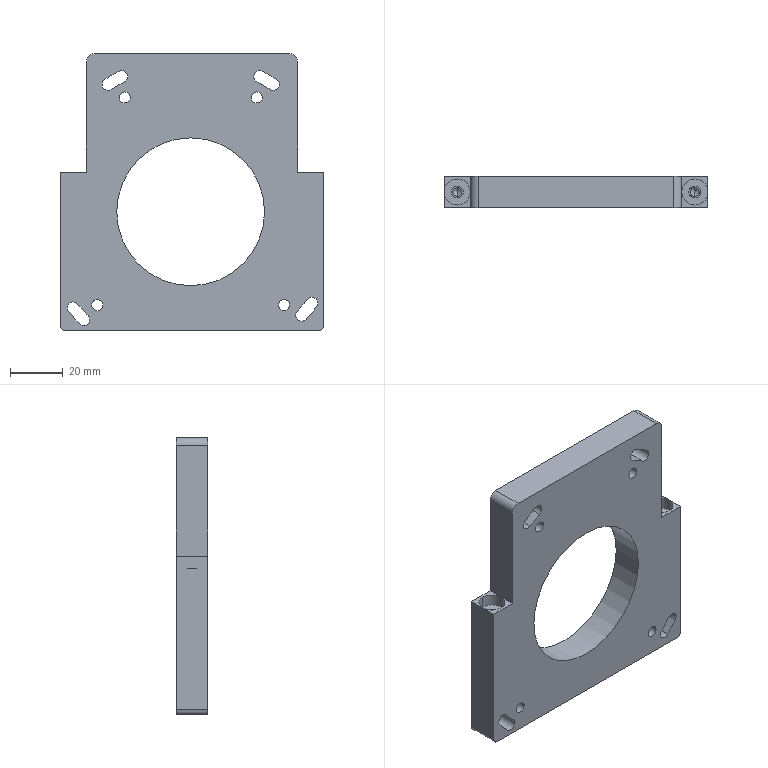CAM job | Mastercam | mm | 14 operations | part box 100 x 11.9 x 105
1. Facing | 24 - 100 平铣刀
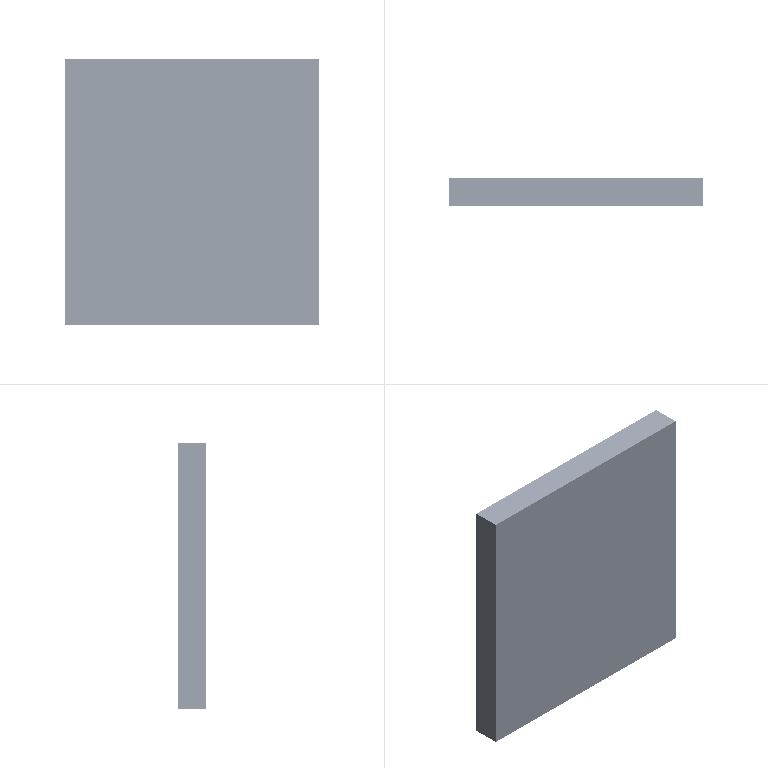2. 2D High Speed (2D Dynamic Mill) | 9 - 10 平铣刀
3. 2D High Speed (2D Dynamic Mill) | 9 - 10 平铣刀
4. Contour (Ramp) | 3 - 3 平铣刀
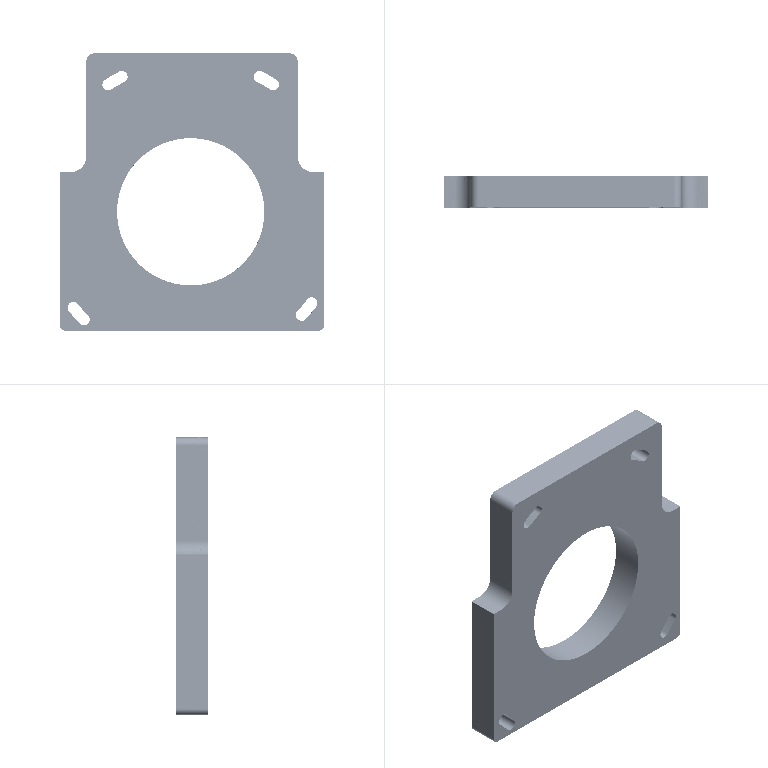5. Contour (Ramp) | 3 - 3 平铣刀
6. Contour (2D) | 10 - 10 平铣刀
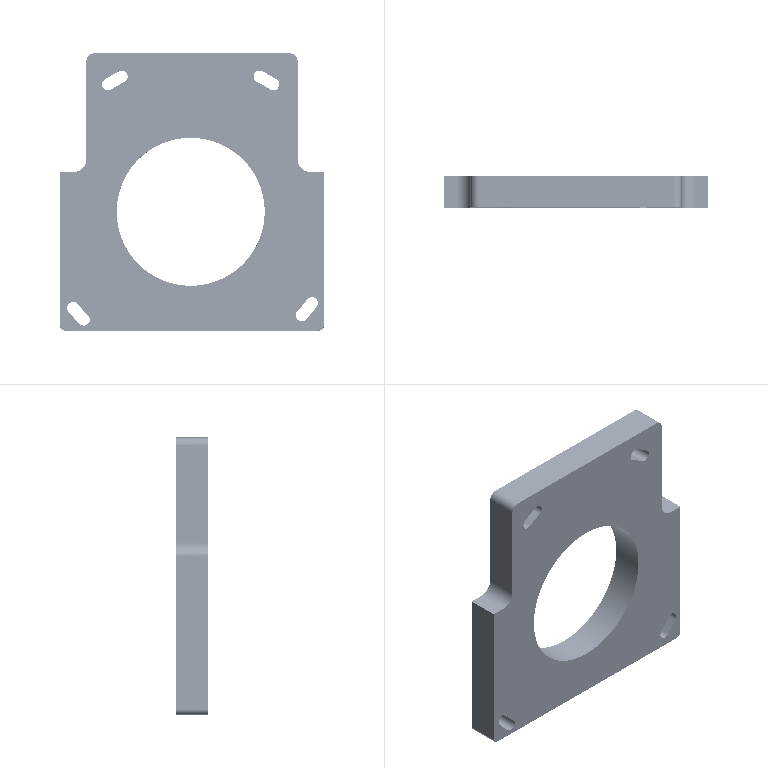7. Contour (2D chamfer) | 5 - 4 倒角刀
8. Facing | 24 - 100 平铣刀
9. Contour (2D chamfer) | 5 - 4 倒角刀
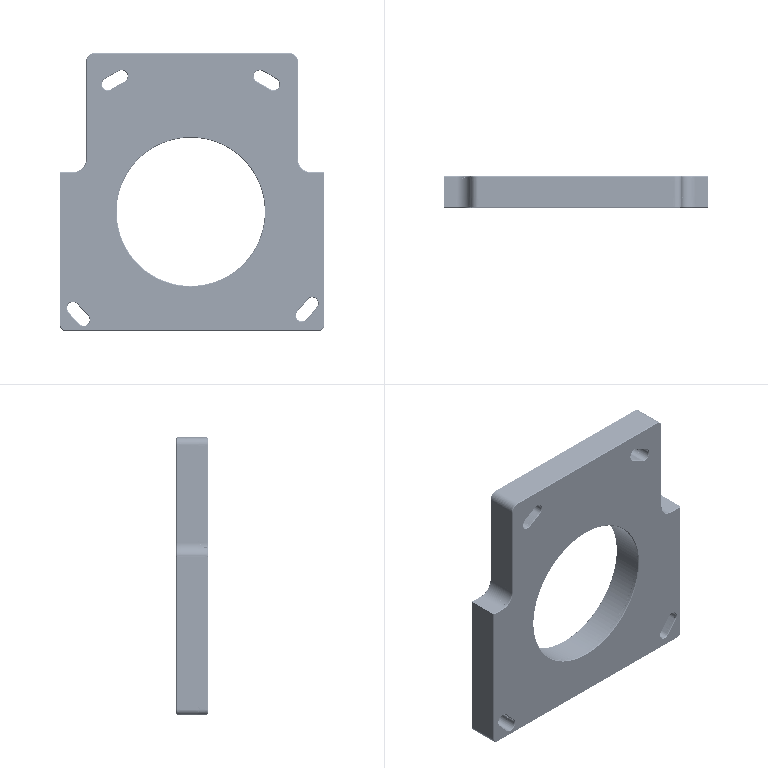10. Contour (Ramp) | 9 - 10 平铣刀
11. Contour (2D) | 10 - 10 平铣刀
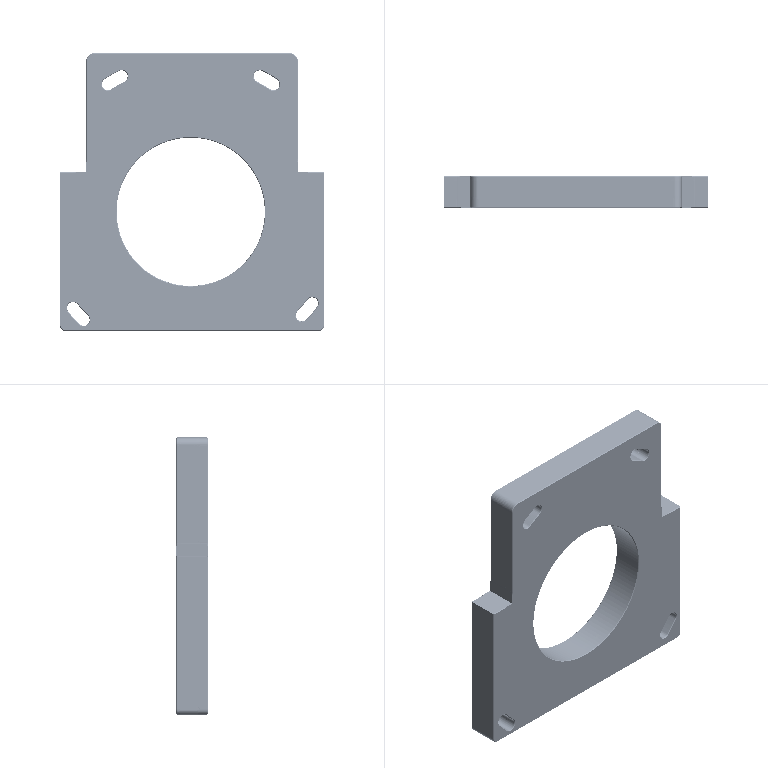12. Contour (Ramp) | 6 - 6 平铣刀
13. Contour (2D) | 6 - 6 平铣刀
14. Drill/Counterbore | 17 - 6 倒角刀